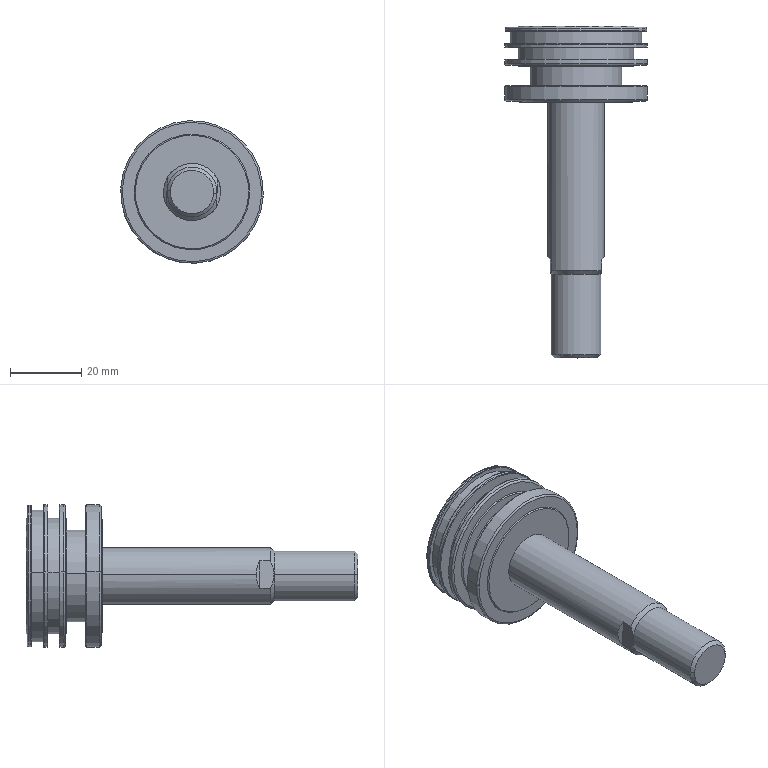Component | SolidWorks | ACQ40x30SB(0)+()-1_ACQS-40x30-B_30r-1 | 1 solid | 60 faces | box 40 x 93 x 40 mm | volume 33590 mm3 | cylinder 18 | plane 16 | torus 14 | cone 12 | commonest cylinder face diameters 40 x6 14 x2 39.6 x2 37 x2 32.4 x2 25.8 x2 16 x2
build123d program:
from build123d import *

# Parameters (mm, degrees)
CUT_EXTRUDE1_DEPTH      = 14
CUT_EXTRUDE1_DEPTH_BACK = 14


with BuildPart() as part:
    # Sketch1 → Revolve1 (revolve)
    with BuildSketch(Plane.XY, mode=Mode.PRIVATE) as revolve1_sk:
        with BuildLine():
            Line((0, 0), (0, 8))
            Line((0, 8), (43.2, 8))
            Line((43.2, 8), (43.2, 15.9))
            Line((43.2, 15.9), (43.5, 16.2))
            Line((43.5, 16.2), (43.5, 19.5))
            ThreePointArc((43.5, 19.5), (43.646, 19.854), (44, 20))
            Line((44, 20), (47.6, 20))
            Line((47.6, 20), (47.8, 19.8))
            Line((47.8, 19.8), (47.8, 12.9))
            Line((47.8, 12.9), (53.2, 12.9))
            Line((53.2, 12.9), (53.2, 16.2))
            Line((53.2, 16.2), (53.5, 16.5))
            Line((53.5, 16.5), (53.5, 19.5))
            ThreePointArc((53.5, 19.5), (53.646, 19.854), (54, 20))
            Line((54, 20), (55, 20))
            ThreePointArc((55, 20), (55.141, 19.941), (55.2, 19.8))
            Line((55.2, 19.8), (55.2, 16.2))
            Line((55.2, 16.2), (58.4, 16.2))
            Line((58.4, 16.2), (58.4, 19.8))
            ThreePointArc((58.4, 19.8), (58.459, 19.941), (58.6, 20))
            Line((58.6, 20), (59.4, 20))
            ThreePointArc((59.4, 20), (59.541, 19.941), (59.6, 19.8))
            Line((59.6, 19.8), (59.6, 18.5))
            Line((59.6, 18.5), (63, 18.5))
            Line((63, 18.5), (63, 19.6))
            ThreePointArc((63, 19.6), (63.059, 19.741), (63.2, 19.8))
            Line((63.2, 19.8), (63.7, 19.8))
            ThreePointArc((63.7, 19.8), (64.054, 19.654), (64.2, 19.3))
            Line((64.2, 19.3), (64.2, 16.5))
            Line((64.2, 16.5), (64.5, 16.2))
            Line((64.5, 16.2), (64.5, 0))
            Line((64.5, 0), (0, 0))
        make_face()
    revolve(revolve1_sk.sketch.rotate(Axis((64.5, 0, 0), (-1, 0, 0)), 270), axis=Axis((64.5, 0, 0), (-1, 0, 0)))

    # Sketch2 → Revolve2 (revolve)
    with BuildSketch(Plane.XY, mode=Mode.PRIVATE) as revolve2_sk:
        Polygon((-28.5, 0), (-28.5, 6.08), (-27.58, 7), (-5, 7), (-4, 8), (0, 8), (0, 0), align=None)
    revolve(revolve2_sk.sketch.rotate(Axis((0, 0, 0), (-1, 0, 0)), 270), axis=Axis((0, 0, 0), (-1, 0, 0)))

    # Sketch3 → Cut-Extrude1 (cut, two sides: drawn at the far end of the back side and taken through both)
    with BuildSketch(Plane(origin=(0, 0, 0), x_dir=(1, 0, 0), z_dir=(0, 1, 0)).offset(-CUT_EXTRUDE1_DEPTH_BACK)):
        Polygon((-38.5, 27), (-38.5, -27), (19, -27), (-1, -7), (-5, -7), (-5, -15), (-28.5, -15), (-28.5, 15), (-5, 15), (-5, 7), (-1, 7), (19, 27), align=None)
    extrude(amount=CUT_EXTRUDE1_DEPTH + CUT_EXTRUDE1_DEPTH_BACK, mode=Mode.SUBTRACT)


solid = part.part

# Placed as in the assembly
solid = solid.moved(Location((-28.439, -45.745, 290), (180, 86.737, -90)))